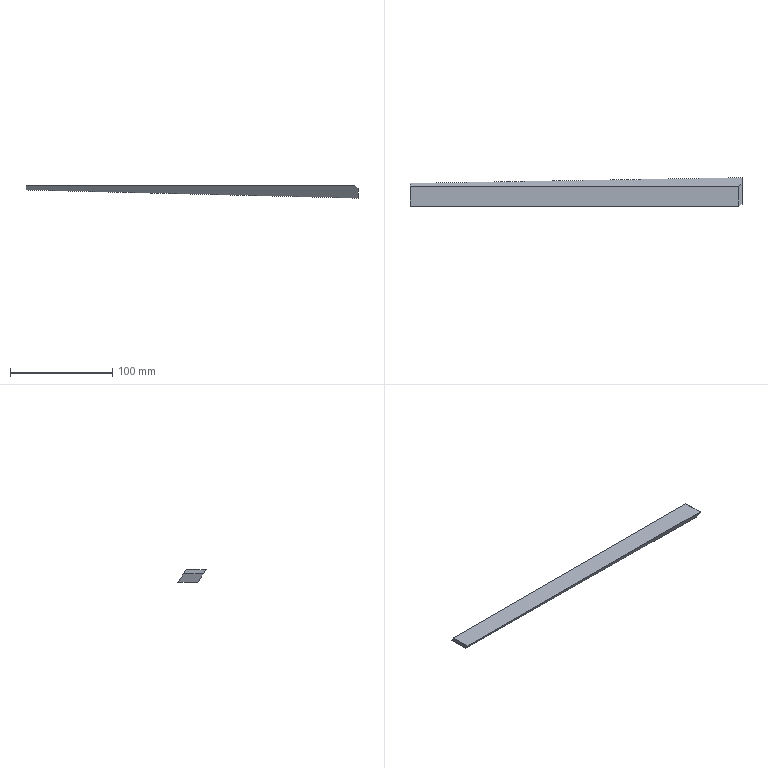Component | SolidWorks | 19Insert-1 | 1 solid | 7 faces | box 325 x 27.93 x 12 mm | volume 50696 mm3 | plane 7
build123d program:
from build123d import *

# Parameters (mm, degrees)
BOSS_EXTRUDE1_DEPTH     = 30
CHAMFER1_SIZE           = 3
CUT_EXTRUDE1_DEPTH      = 327.602
CUT_EXTRUDE1_DEPTH_BACK = 327.602


with BuildPart() as part:
    # Sketch1 → Boss-Extrude1 (new body)
    with BuildSketch(Plane.XY):
        Polygon((0, 0), (325, 8), (325, 12), (0, 12), align=None)
    extrude(amount=BOSS_EXTRUDE1_DEPTH)

    # Chamfer1
    chamfer1_edges = [part.edges().sort_by_distance(p)[0] for p in [
        (0, 12, 15),
    ]]
    chamfer(chamfer1_edges, length=CHAMFER1_SIZE)

    # Sketch2 → Cut-Extrude1 (cut, two sides: drawn at the far end of the back side and taken through both)
    with BuildSketch(Plane.ZY.offset(-CUT_EXTRUDE1_DEPTH_BACK)):
        Polygon((10.468, 0), (4.166, 9), (0, 9), (0, 0), align=None)
        Polygon((30, 9), (23.698, 9), (30, 0), align=None)
        Polygon((21.598, 12), (23.698, 9), (30, 9), (30, 0), (32.608, 12), align=None)
        Polygon((4.166, 9), (2.065, 12), (0, 12), (0, 9), align=None)
    extrude(amount=CUT_EXTRUDE1_DEPTH + CUT_EXTRUDE1_DEPTH_BACK, mode=Mode.SUBTRACT)


solid = part.part

# Placed as in the assembly
solid = solid.moved(Location((125, 62.935, -92), (-90, 0, 180)))
STEP:
#1=COLOUR_RGB('',0.7922,0.8196,0.9333);
#2=FILL_AREA_STYLE_COLOUR('',#1);
#3=FILL_AREA_STYLE('',(#2));
#4=SURFACE_STYLE_FILL_AREA(#3);
#5=SURFACE_SIDE_STYLE('',(#4));
#6=SURFACE_STYLE_USAGE(.BOTH.,#5);
#7=PRESENTATION_STYLE_ASSIGNMENT((#6));
#8=CARTESIAN_POINT('',(4.921,3.659,-3.622));
#9=VERTEX_POINT('',#8);
#10=CARTESIAN_POINT('',(4.921,2.89,-3.622));
#11=VERTEX_POINT('',#10);
#12=CARTESIAN_POINT('',(4.921,3.659,-3.622));
#13=DIRECTION('',(-0.,-1.,0.));
#14=VECTOR('',#13,39.37);
#15=LINE('',#12,#14);
#16=EDGE_CURVE('',#9,#11,#15,.T.);
#17=ORIENTED_EDGE('',*,*,#16,.F.);
#18=CARTESIAN_POINT('',(4.921,3.411,-3.268));
#19=VERTEX_POINT('',#18);
#20=CARTESIAN_POINT('',(4.921,3.437,-3.305));
#21=DIRECTION('',(-0.,-0.5736,0.8192));
#22=VECTOR('',#21,39.37);
#23=LINE('',#20,#22);
#24=EDGE_CURVE('',#9,#19,#23,.T.);
#25=ORIENTED_EDGE('',*,*,#24,.T.);
#26=CARTESIAN_POINT('',(4.921,2.642,-3.268));
#27=VERTEX_POINT('',#26);
#28=CARTESIAN_POINT('',(4.921,3.659,-3.268));
#29=DIRECTION('',(-0.,-1.,0.));
#30=VECTOR('',#29,39.37);
#31=LINE('',#28,#30);
#32=EDGE_CURVE('',#19,#27,#31,.T.);
#33=ORIENTED_EDGE('',*,*,#32,.T.);
#34=CARTESIAN_POINT('',(4.921,2.921,-3.666));
#35=DIRECTION('',(-0.,-0.5736,0.8192));
#36=VECTOR('',#35,39.37);
#37=LINE('',#34,#36);
#38=EDGE_CURVE('',#11,#27,#37,.T.);
#39=ORIENTED_EDGE('',*,*,#38,.F.);
#40=EDGE_LOOP('',(#17,#25,#33,#39));
#41=FACE_OUTER_BOUND('',#40,.T.);
#42=CARTESIAN_POINT('',(4.921,3.659,-3.15));
#43=DIRECTION('',(-1.,0.,0.));
#44=DIRECTION('',(0.,0.,1.));
#45=AXIS2_PLACEMENT_3D('',#42,#43,#44);
#46=PLANE('',#45);
#47=ADVANCED_FACE('',(#41),#46,.F.);
#48=CARTESIAN_POINT('',(-7.874,3.438,-3.307));
#49=VERTEX_POINT('',#48);
#50=CARTESIAN_POINT('',(-7.874,2.669,-3.307));
#51=VERTEX_POINT('',#50);
#52=CARTESIAN_POINT('',(-7.874,3.659,-3.307));
#53=DIRECTION('',(-0.,-1.,0.));
#54=VECTOR('',#53,39.37);
#55=LINE('',#52,#54);
#56=EDGE_CURVE('',#49,#51,#55,.T.);
#57=ORIENTED_EDGE('',*,*,#56,.F.);
#58=CARTESIAN_POINT('',(4.921,3.659,-3.622));
#59=DIRECTION('',(0.9995,0.01723,-0.0246));
#60=VECTOR('',#59,39.37);
#61=LINE('',#58,#60);
#62=EDGE_CURVE('',#49,#9,#61,.T.);
#63=ORIENTED_EDGE('',*,*,#62,.T.);
#64=ORIENTED_EDGE('',*,*,#16,.T.);
#65=CARTESIAN_POINT('',(4.935,2.89,-3.622));
#66=DIRECTION('',(0.9995,0.01723,-0.0246));
#67=VECTOR('',#66,39.37);
#68=LINE('',#65,#67);
#69=EDGE_CURVE('',#51,#11,#68,.T.);
#70=ORIENTED_EDGE('',*,*,#69,.F.);
#71=EDGE_LOOP('',(#57,#63,#64,#70));
#72=FACE_OUTER_BOUND('',#71,.T.);
#73=CARTESIAN_POINT('',(4.921,3.659,-3.622));
#74=DIRECTION('',(0.02461,0.,0.9997));
#75=DIRECTION('',(0.9997,-0.,-0.02461));
#76=AXIS2_PLACEMENT_3D('',#73,#74,#75);
#77=PLANE('',#76);
#78=ADVANCED_FACE('',(#72),#77,.F.);
#79=CARTESIAN_POINT('',(-7.874,3.328,-3.15));
#80=VERTEX_POINT('',#79);
#81=CARTESIAN_POINT('',(-7.874,2.559,-3.15));
#82=VERTEX_POINT('',#81);
#83=CARTESIAN_POINT('',(-7.874,3.659,-3.15));
#84=DIRECTION('',(-0.,-1.,0.));
#85=VECTOR('',#84,39.37);
#86=LINE('',#83,#85);
#87=EDGE_CURVE('',#80,#82,#86,.T.);
#88=ORIENTED_EDGE('',*,*,#87,.F.);
#89=CARTESIAN_POINT('',(-7.874,3.27,-3.067));
#90=DIRECTION('',(0.,0.5736,-0.8192));
#91=VECTOR('',#90,39.37);
#92=LINE('',#89,#91);
#93=EDGE_CURVE('',#80,#49,#92,.T.);
#94=ORIENTED_EDGE('',*,*,#93,.T.);
#95=ORIENTED_EDGE('',*,*,#56,.T.);
#96=CARTESIAN_POINT('',(-7.874,2.754,-3.428));
#97=DIRECTION('',(0.,0.5736,-0.8192));
#98=VECTOR('',#97,39.37);
#99=LINE('',#96,#98);
#100=EDGE_CURVE('',#82,#51,#99,.T.);
#101=ORIENTED_EDGE('',*,*,#100,.F.);
#102=EDGE_LOOP('',(#88,#94,#95,#101));
#103=FACE_OUTER_BOUND('',#102,.T.);
#104=CARTESIAN_POINT('',(-7.874,3.659,-3.307));
#105=DIRECTION('',(1.,-0.,0.));
#106=DIRECTION('',(0.,1.,-0.));
#107=AXIS2_PLACEMENT_3D('',#104,#105,#106);
#108=PLANE('',#107);
#109=ADVANCED_FACE('',(#103),#108,.F.);
#110=CARTESIAN_POINT('',(4.803,2.559,-3.15));
#111=VERTEX_POINT('',#110);
#112=CARTESIAN_POINT('',(4.803,3.328,-3.15));
#113=VERTEX_POINT('',#112);
#114=CARTESIAN_POINT('',(4.803,3.659,-3.15));
#115=DIRECTION('',(0.,1.,-0.));
#116=VECTOR('',#115,39.37);
#117=LINE('',#114,#116);
#118=EDGE_CURVE('',#111,#113,#117,.T.);
#119=ORIENTED_EDGE('',*,*,#118,.T.);
#120=CARTESIAN_POINT('',(-7.874,3.328,-3.15));
#121=DIRECTION('',(1.,-0.,-0.));
#122=VECTOR('',#121,39.37);
#123=LINE('',#120,#122);
#124=EDGE_CURVE('',#80,#113,#123,.T.);
#125=ORIENTED_EDGE('',*,*,#124,.F.);
#126=ORIENTED_EDGE('',*,*,#87,.T.);
#127=CARTESIAN_POINT('',(-7.874,2.559,-3.15));
#128=DIRECTION('',(1.,-0.,-0.));
#129=VECTOR('',#128,39.37);
#130=LINE('',#127,#129);
#131=EDGE_CURVE('',#82,#111,#130,.T.);
#132=ORIENTED_EDGE('',*,*,#131,.T.);
#133=EDGE_LOOP('',(#119,#125,#126,#132));
#134=FACE_OUTER_BOUND('',#133,.T.);
#135=CARTESIAN_POINT('',(-7.874,3.659,-3.15));
#136=DIRECTION('',(-0.,-0.,-1.));
#137=DIRECTION('',(-1.,0.,0.));
#138=AXIS2_PLACEMENT_3D('',#135,#136,#137);
#139=PLANE('',#138);
#140=ADVANCED_FACE('',(#134),#139,.F.);
#141=CARTESIAN_POINT('',(4.991,3.46,-3.337));
#142=DIRECTION('',(0.6337,0.4437,-0.6337));
#143=VECTOR('',#142,39.37);
#144=LINE('',#141,#143);
#145=EDGE_CURVE('',#113,#19,#144,.T.);
#146=ORIENTED_EDGE('',*,*,#145,.F.);
#147=ORIENTED_EDGE('',*,*,#118,.F.);
#148=CARTESIAN_POINT('',(5.207,2.842,-3.554));
#149=DIRECTION('',(0.6337,0.4437,-0.6337));
#150=VECTOR('',#149,39.37);
#151=LINE('',#148,#150);
#152=EDGE_CURVE('',#111,#27,#151,.T.);
#153=ORIENTED_EDGE('',*,*,#152,.T.);
#154=ORIENTED_EDGE('',*,*,#32,.F.);
#155=EDGE_LOOP('',(#146,#147,#153,#154));
#156=FACE_OUTER_BOUND('',#155,.T.);
#157=CARTESIAN_POINT('',(4.921,3.659,-3.268));
#158=DIRECTION('',(-0.7071,-0.,-0.7071));
#159=DIRECTION('',(-0.,-1.,0.));
#160=AXIS2_PLACEMENT_3D('',#157,#158,#159);
#161=PLANE('',#160);
#162=ADVANCED_FACE('',(#156),#161,.F.);
#163=ORIENTED_EDGE('',*,*,#69,.T.);
#164=ORIENTED_EDGE('',*,*,#38,.T.);
#165=ORIENTED_EDGE('',*,*,#152,.F.);
#166=ORIENTED_EDGE('',*,*,#131,.F.);
#167=ORIENTED_EDGE('',*,*,#100,.T.);
#168=EDGE_LOOP('',(#163,#164,#165,#166,#167));
#169=FACE_OUTER_BOUND('',#168,.T.);
#170=CARTESIAN_POINT('',(-7.874,2.754,-3.428));
#171=DIRECTION('',(-0.,-0.8192,-0.5736));
#172=DIRECTION('',(-0.,-0.5736,0.8192));
#173=AXIS2_PLACEMENT_3D('',#170,#171,#172);
#174=PLANE('',#173);
#175=ADVANCED_FACE('',(#169),#174,.T.);
#176=ORIENTED_EDGE('',*,*,#93,.F.);
#177=ORIENTED_EDGE('',*,*,#124,.T.);
#178=ORIENTED_EDGE('',*,*,#145,.T.);
#179=ORIENTED_EDGE('',*,*,#24,.F.);
#180=ORIENTED_EDGE('',*,*,#62,.F.);
#181=EDGE_LOOP('',(#176,#177,#178,#179,#180));
#182=FACE_OUTER_BOUND('',#181,.T.);
#183=CARTESIAN_POINT('',(-7.874,3.27,-3.067));
#184=DIRECTION('',(-0.,-0.8192,-0.5736));
#185=DIRECTION('',(-0.,-0.5736,0.8192));
#186=AXIS2_PLACEMENT_3D('',#183,#184,#185);
#187=PLANE('',#186);
#188=ADVANCED_FACE('',(#182),#187,.F.);
#189=CLOSED_SHELL('',(#47,#78,#109,#140,#162,#175,#188));
#190=MANIFOLD_SOLID_BREP('',#189);
#191=STYLED_ITEM('',(#7),#190);
#192=(LENGTH_UNIT()NAMED_UNIT(*)SI_UNIT($,.METRE.));
#193=LENGTH_MEASURE_WITH_UNIT(LENGTH_MEASURE(0.0254),#192);
#194=DIMENSIONAL_EXPONENTS(1.,0.,0.,0.,0.,0.,0.);
#195=(CONVERSION_BASED_UNIT('',#193)LENGTH_UNIT()NAMED_UNIT(#194));
#196=UNCERTAINTY_MEASURE_WITH_UNIT(LENGTH_MEASURE(0.00001),#195,'','');
#197=(NAMED_UNIT(*)PLANE_ANGLE_UNIT()SI_UNIT($,.RADIAN.));
#198=(NAMED_UNIT(*)SI_UNIT($,.STERADIAN.)SOLID_ANGLE_UNIT());
#199=(GEOMETRIC_REPRESENTATION_CONTEXT(3)GLOBAL_UNCERTAINTY_ASSIGNED_CONTEXT((#196))GLOBAL_UNIT_ASSIGNED_CONTEXT((#195,#197,#198))REPRESENTATION_CONTEXT('',''));
#200=MECHANICAL_DESIGN_GEOMETRIC_PRESENTATION_REPRESENTATION('',(#191),#199);
#201=PRESENTATION_LAYER_ASSIGNMENT('','',(#191));
#202=CARTESIAN_POINT('',(0.,0.,0.));
#203=DIRECTION('',(0.,0.,1.));
#204=DIRECTION('',(1.,0.,0.));
#205=AXIS2_PLACEMENT_3D('',#202,#203,#204);
#206=(LENGTH_UNIT()NAMED_UNIT(*)SI_UNIT($,.METRE.));
#207=LENGTH_MEASURE_WITH_UNIT(LENGTH_MEASURE(0.0254),#206);
#208=DIMENSIONAL_EXPONENTS(1.,0.,0.,0.,0.,0.,0.);
#209=(CONVERSION_BASED_UNIT('',#207)LENGTH_UNIT()NAMED_UNIT(#208));
#210=UNCERTAINTY_MEASURE_WITH_UNIT(LENGTH_MEASURE(0.00001),#209,'','');
#211=(NAMED_UNIT(*)PLANE_ANGLE_UNIT()SI_UNIT($,.RADIAN.));
#212=(NAMED_UNIT(*)SI_UNIT($,.STERADIAN.)SOLID_ANGLE_UNIT());
#213=(GEOMETRIC_REPRESENTATION_CONTEXT(3)GLOBAL_UNCERTAINTY_ASSIGNED_CONTEXT((#210))GLOBAL_UNIT_ASSIGNED_CONTEXT((#209,#211,#212))REPRESENTATION_CONTEXT('',''));
#214=ADVANCED_BREP_SHAPE_REPRESENTATION('',(#190,#205),#213);